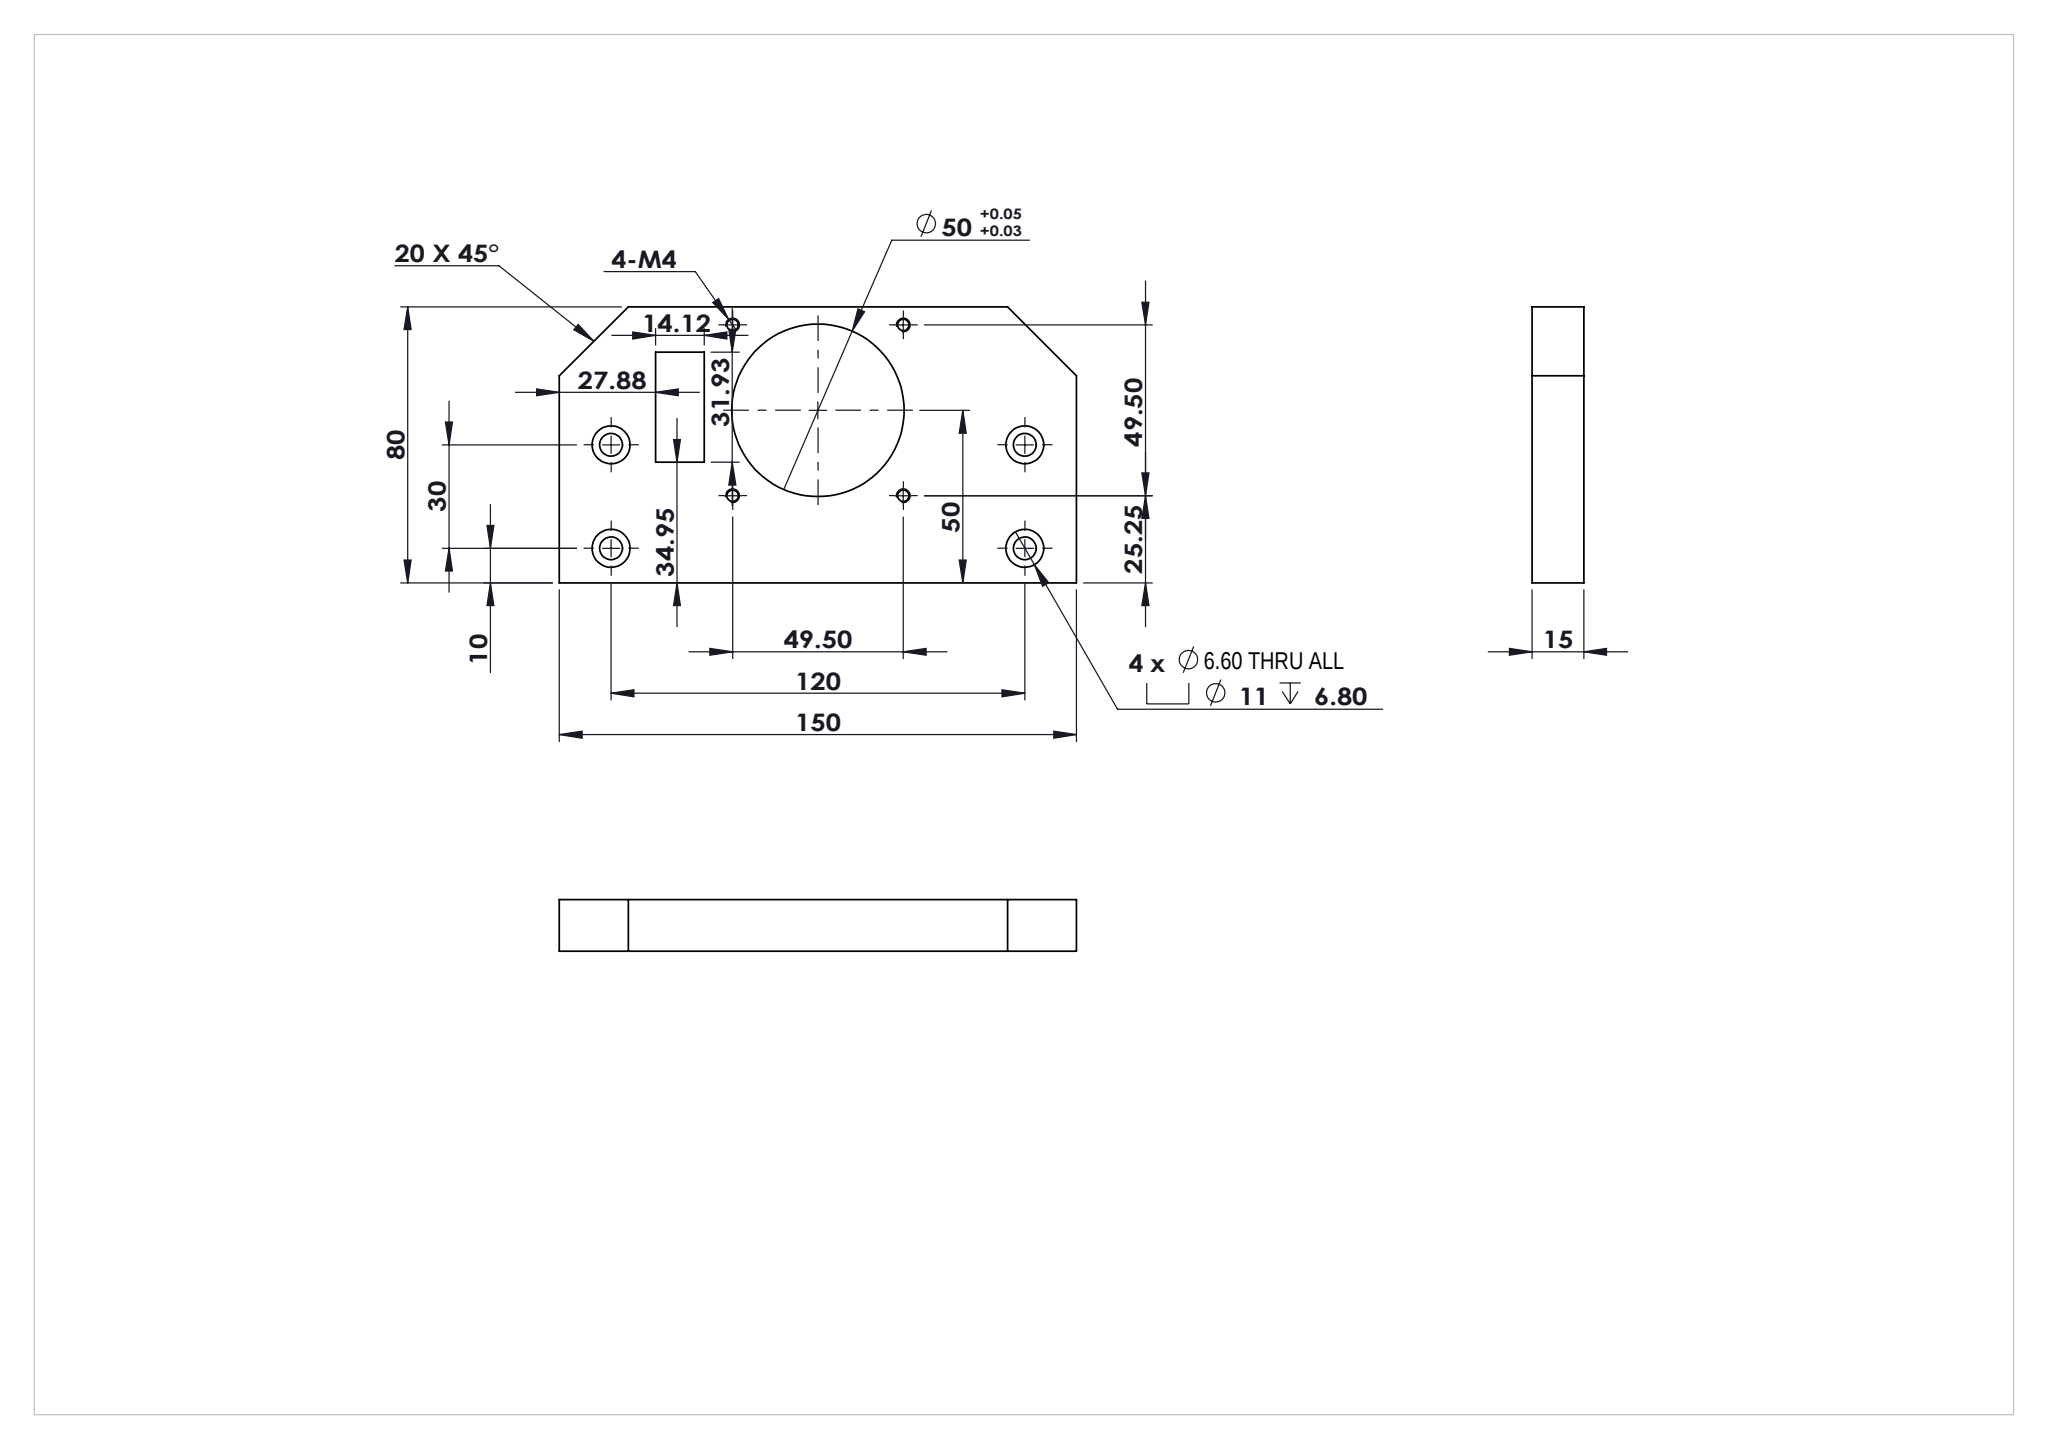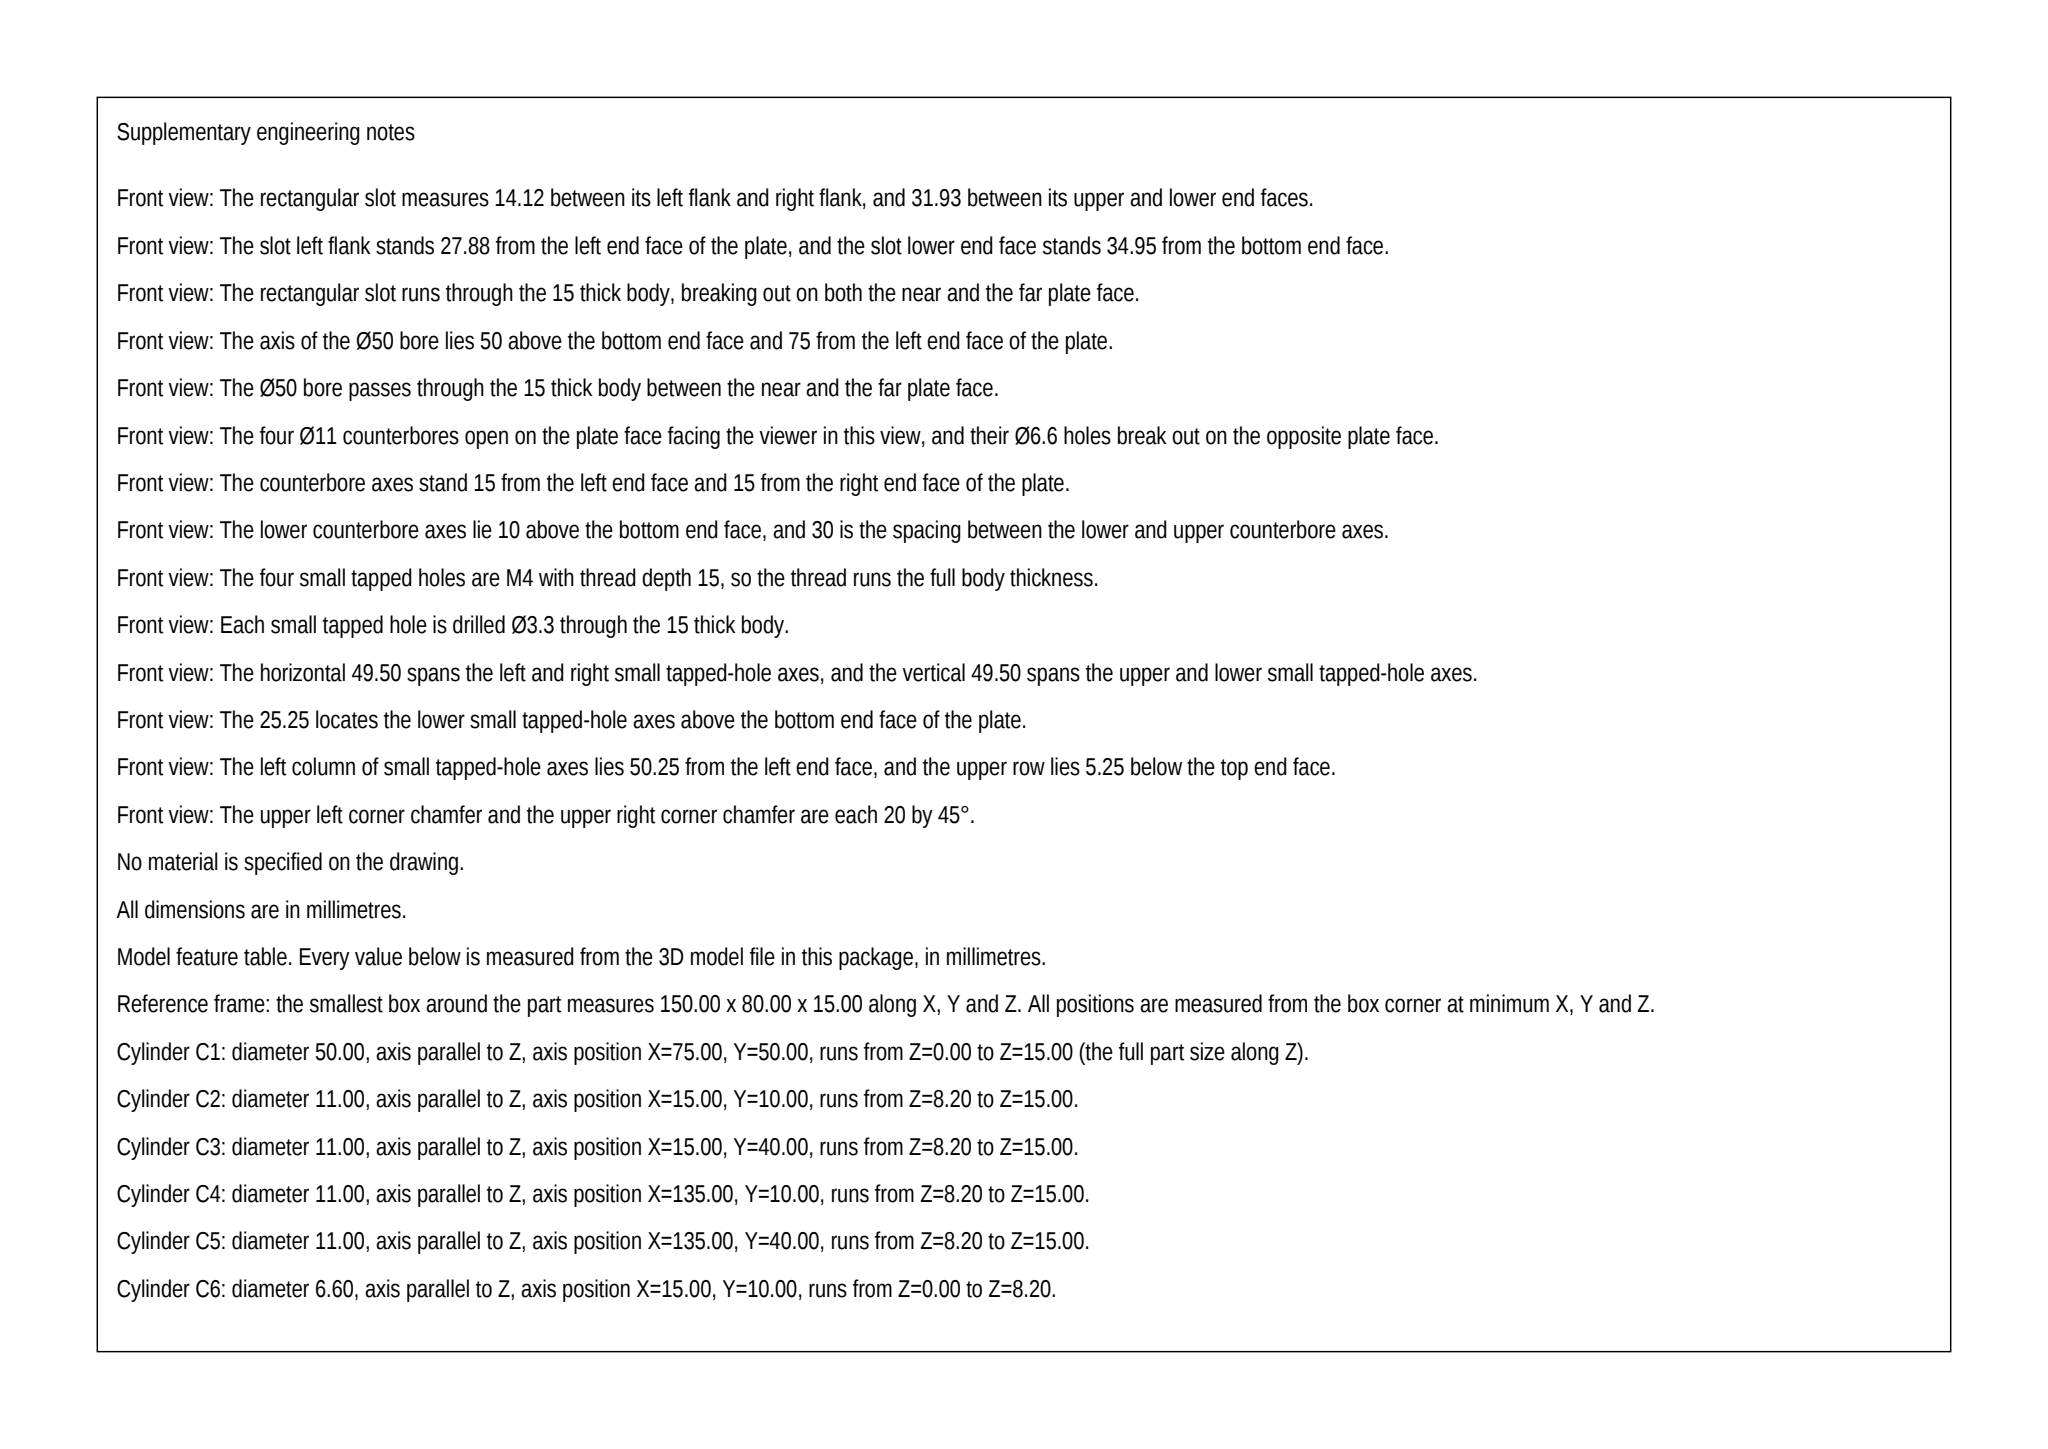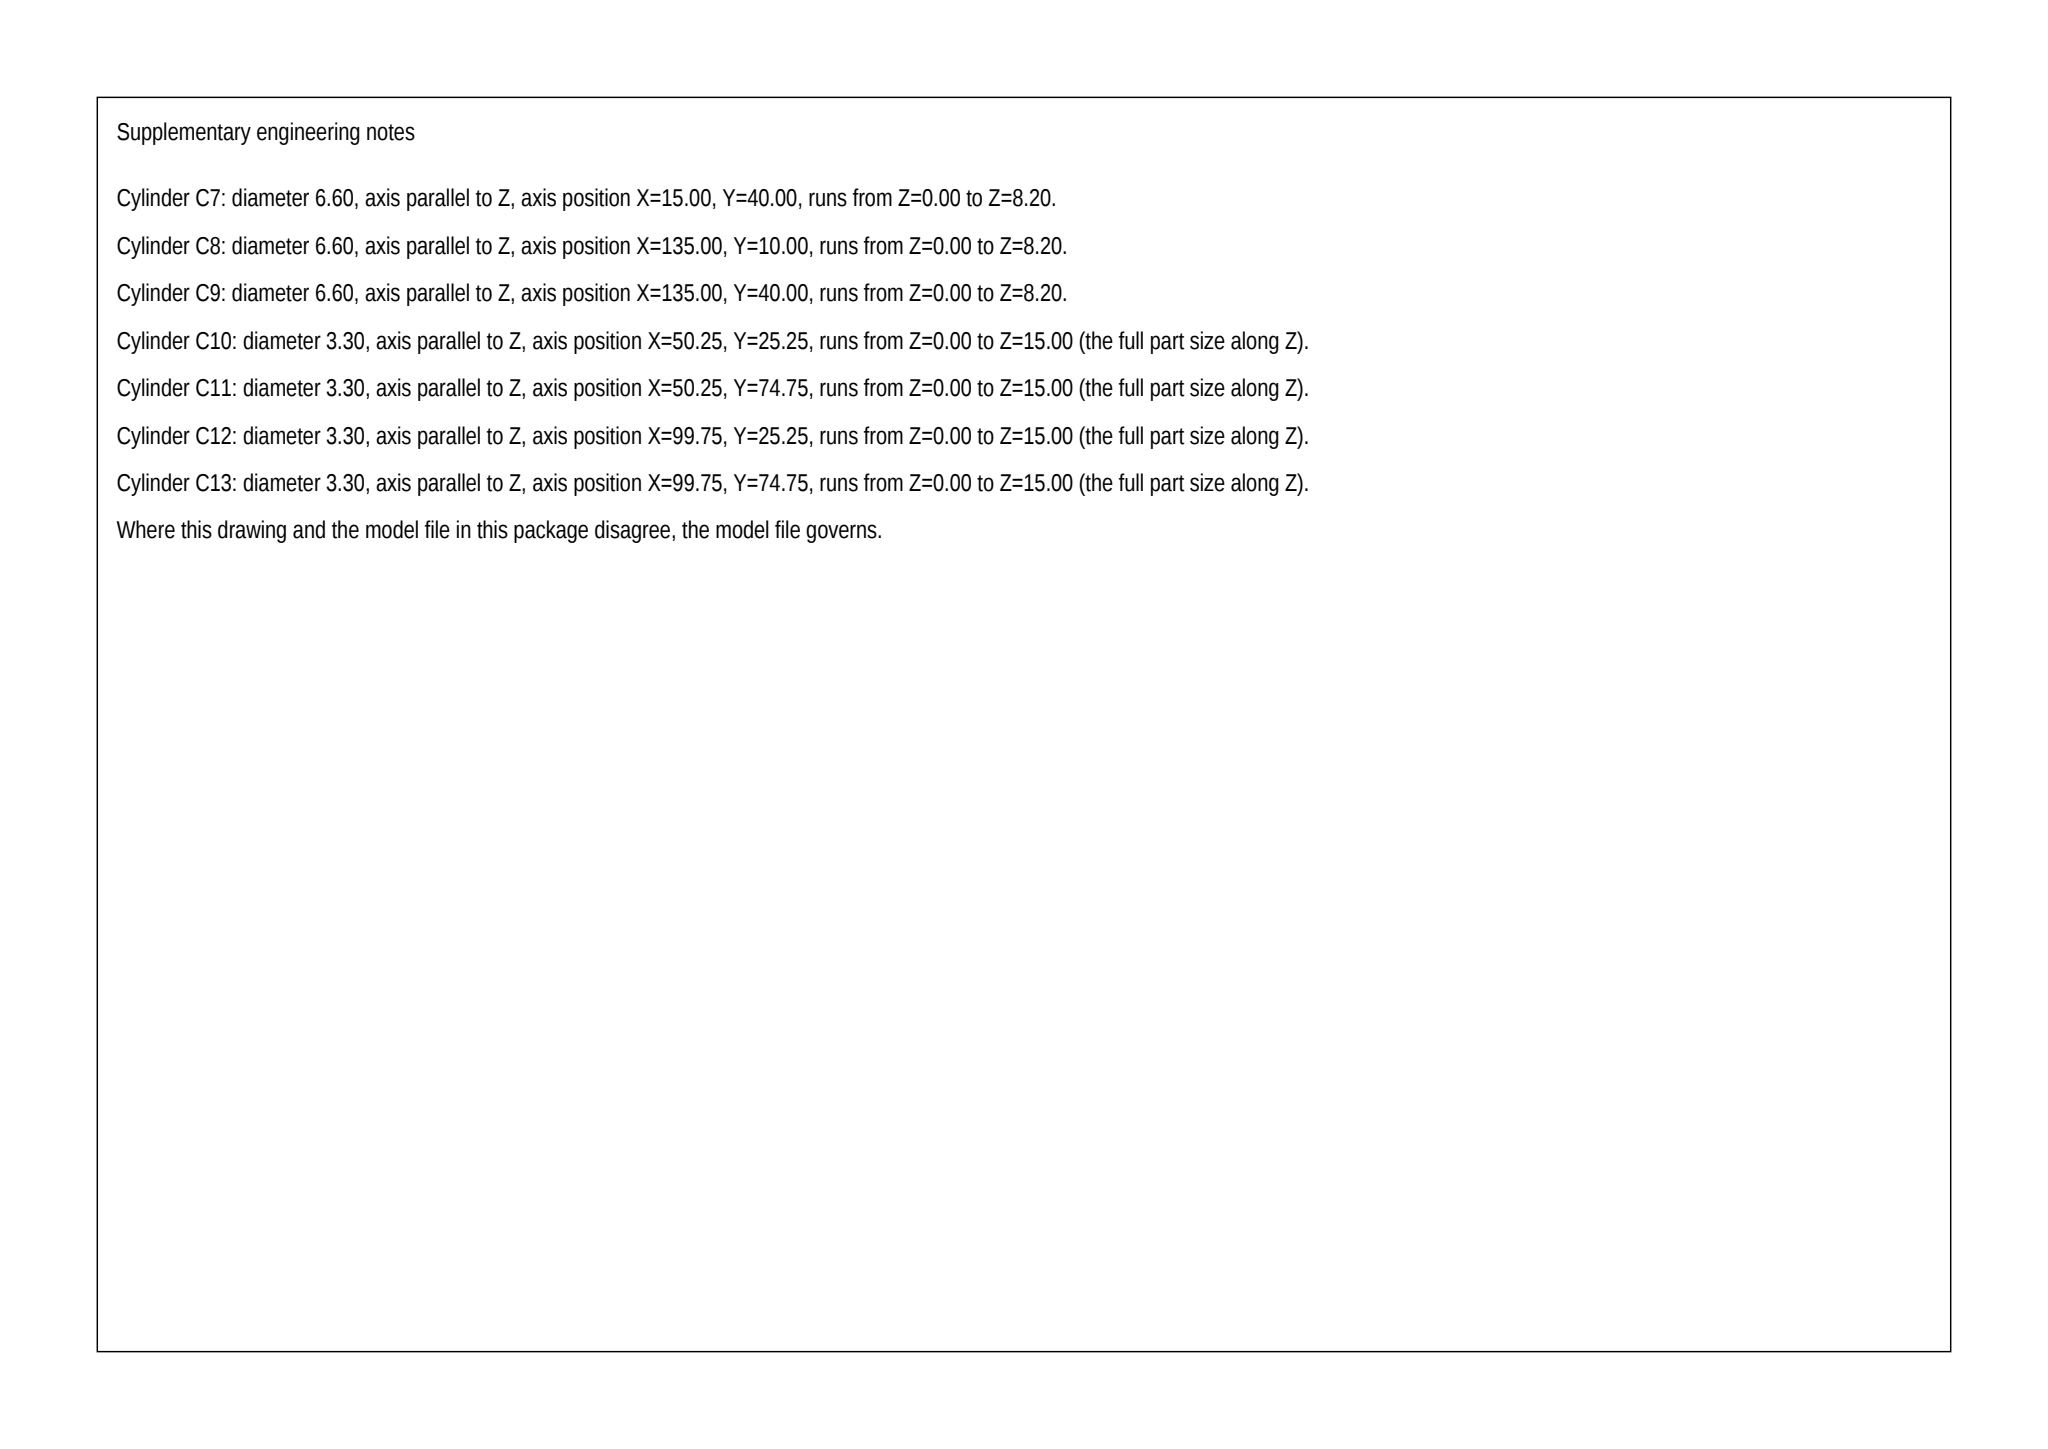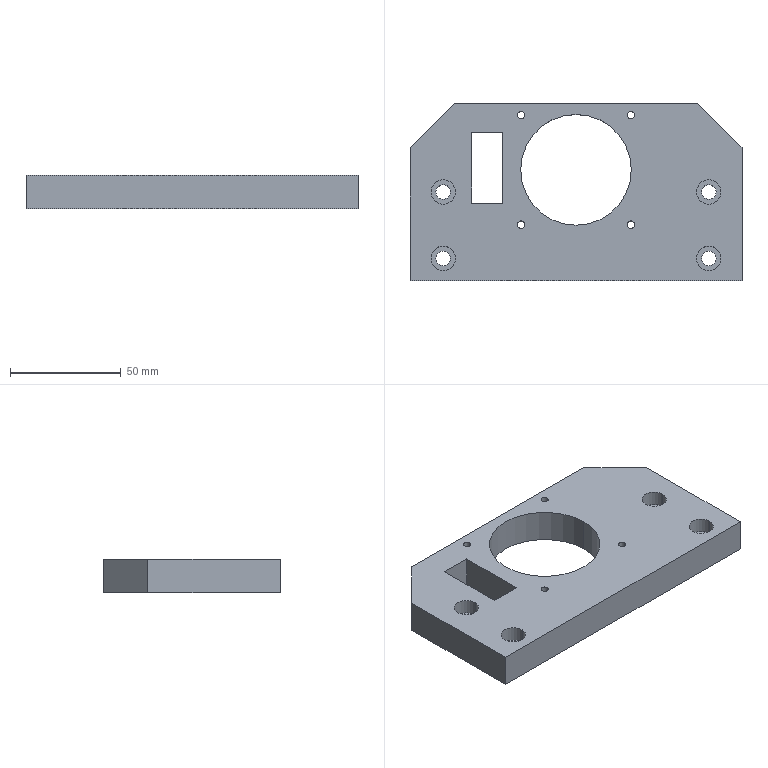Part | SolidWorks | mm | 1 solid | 42 faces | box 150 x 80 x 15 mm | volume 133563 mm3 | cylinder 26 | plane 16 | commonest cylinder face diameters 11 x8 6.6 x8 3.3 x8 50 x2
Drawing notes:
RECT SLOT 14.12 X 31.93 THRU (15 THK) | from the solid: Planes x=27.88 & x=42.0 (14.12 wide), y=34.95 & y=66.88 (31.93); no intermediate z plane within slot, bbox thk 15.0 -> cut full depth
build123d program:
from build123d import *

# Parameters (mm, degrees)
SKETCH1_2_W                                          = 150
SKETCH1_2_H                                          = 80
BOSS_EXTRUDE1_DEPTH                                  = 15
SKETCH3_2_R                                          = 25
CUT_EXTRUDE1_DEPTH                                   = 87.313
CHAMFER1_SIZE                                        = 20
M4_TAPPED_HOLE1_D                                    = 3.3
CBORE_FOR_M6_HEXAGON_SOCKET_HEAD_CAP_SCR_D           = 6.6
CBORE_FOR_M6_HEXAGON_SOCKET_HEAD_CAP_SCR_CBORE_D     = 11
CBORE_FOR_M6_HEXAGON_SOCKET_HEAD_CAP_SCR_CBORE_DEPTH = 6.8
SKETCH4_2_W                                          = 14.124
SKETCH4_2_H                                          = 31.928
CUT_EXTRUDE2_DEPTH                                   = 45


with BuildPart() as part:
    # Sketch1_2 → Boss-Extrude1 (new body)
    with BuildSketch(Plane.XY):
        Rectangle(SKETCH1_2_W, SKETCH1_2_H)
    extrude(amount=BOSS_EXTRUDE1_DEPTH)

    # Sketch3_2 → Cut-Extrude1 (cut, through all)
    with BuildSketch(Plane.XY.offset(15)):
        with Locations((0, 10)):
            Circle(SKETCH3_2_R)
    extrude(amount=-CUT_EXTRUDE1_DEPTH, mode=Mode.SUBTRACT)

    # Chamfer1
    chamfer1_edges = [part.edges().sort_by_distance(p)[0] for p in [
        (-75, 40, 7.5),
        (75, 40, 7.5),
    ]]
    chamfer(chamfer1_edges, length=CHAMFER1_SIZE)

    # M4 Tapped Hole1 (through all)
    with Locations(Plane.XY.offset(15)):
        with Locations((-24.749, 34.749), (-24.749, -14.749), (24.749, -14.749), (24.749, 34.749)):
            Hole(M4_TAPPED_HOLE1_D / 2)

    # CBORE for M6 Hexagon socket head cap scr (through all)
    with Locations(Plane.XY.offset(15)):
        with Locations((-60, 0), (-60, -30), (60, -30), (60, 0)):
            CounterBoreHole(CBORE_FOR_M6_HEXAGON_SOCKET_HEAD_CAP_SCR_D / 2, CBORE_FOR_M6_HEXAGON_SOCKET_HEAD_CAP_SCR_CBORE_D / 2, CBORE_FOR_M6_HEXAGON_SOCKET_HEAD_CAP_SCR_CBORE_DEPTH)

    # Sketch4_2 → Cut-Extrude2 (cut)
    with BuildSketch(Plane.XY.offset(15)):
        with Locations((-40.058, 10.913)):
            Rectangle(SKETCH4_2_W, SKETCH4_2_H)
    extrude(amount=-CUT_EXTRUDE2_DEPTH, mode=Mode.SUBTRACT)


solid = part.part